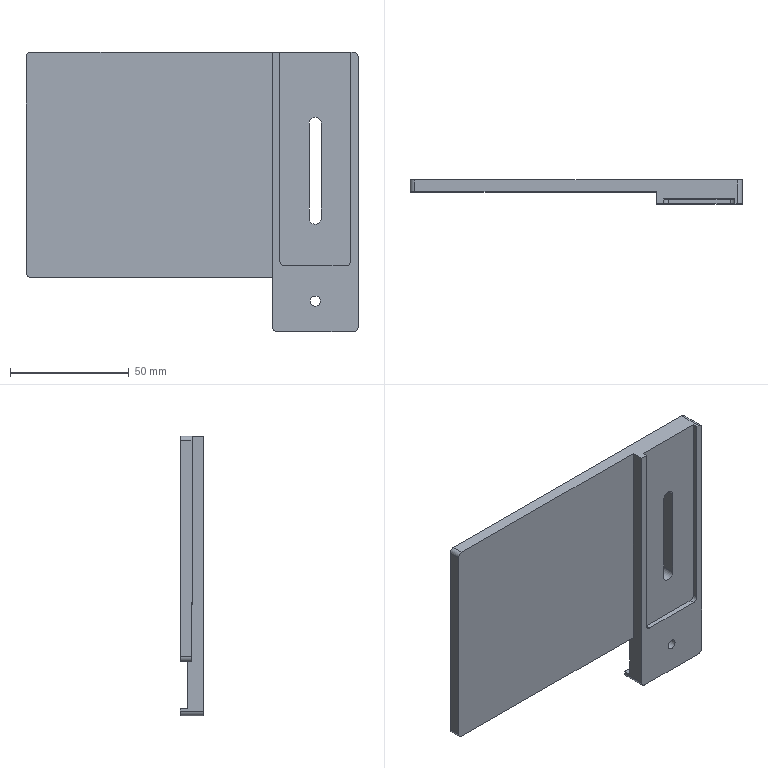Component | SolidWorks | SecondGenerationFour-sidedLabelingTopBatteryPlate-1 | 1 solid | 29 faces | box 140 x 10 x 118 mm | volume 82358 mm3 | plane 18 | cylinder 11 | commonest cylinder face diameters 4 x7 4.2 x2 5.2 x2
build123d program:
from build123d import *

# Parameters (mm, degrees)
SKETCH1_W             = 140
SKETCH1_H             = 95
BOSS_EXTRUDE1_DEPTH   = 10
SKETCH12_W            = 104
SKETCH12_H            = 95
CUT_EXTRUDE2_DEPTH    = 5
CUT_EXTRUDE1_DEPTH    = 86.184
SKETCH13_W            = 36
SKETCH13_H            = 7
BOSS_EXTRUDE3_DEPTH   = 20
M5_TAPPED_HOLE2_D     = 4.2
M5_TAPPED_HOLE2_DEPTH = 20
M5_TAPPED_HOLE2_TIP   = 1.262
SKETCH16_W            = 36
SKETCH16_H            = 10
BOSS_EXTRUDE4_DEPTH   = 3
SKETCH18_W            = 30
SKETCH18_H            = 90
CUT_EXTRUDE4_DEPTH    = 2
FILLET2_R             = 2
FILLET1_R             = 2


with BuildPart() as part:
    # Sketch1 → Boss-Extrude1 (new body)
    with BuildSketch(Plane.XY):
        Rectangle(SKETCH1_W, SKETCH1_H)
    extrude(amount=BOSS_EXTRUDE1_DEPTH)

    # Sketch12 → Cut-Extrude2 (cut)
    with BuildSketch(Plane(origin=(0, 0, 0), x_dir=(-1, 0, 0), z_dir=(0, 0, -1))):
        with Locations((-18, 0)):
            Rectangle(SKETCH12_W, SKETCH12_H)
    extrude(amount=-CUT_EXTRUDE2_DEPTH, mode=Mode.SUBTRACT)

    # Sketch9 → Cut-Extrude1 (cut, through all)
    with BuildSketch(Plane.XY.offset(10)):
        with BuildLine():
            Line((-54.6, -22.5), (-54.6, 17.5))
            ThreePointArc((-54.6, 17.5), (-52, 20.1), (-49.4, 17.5))
            Line((-49.4, 17.5), (-49.4, -22.5))
            ThreePointArc((-49.4, -22.5), (-52, -25.1), (-54.6, -22.5))
        make_face()
    extrude(amount=-CUT_EXTRUDE1_DEPTH, mode=Mode.SUBTRACT)

    # Sketch13 → Boss-Extrude3 (add)
    with BuildSketch(Plane.XZ.offset(47.5)):
        with Locations((-52, 3.5)):
            Rectangle(SKETCH13_W, SKETCH13_H)
    extrude(amount=BOSS_EXTRUDE3_DEPTH)

    # M5 Tapped Hole2
    with Locations(Plane.XY.offset(7)):
        with Locations((-52, -57.5)):
            Hole(M5_TAPPED_HOLE2_D / 2, depth=M5_TAPPED_HOLE2_DEPTH)
            with Locations((0, 0, -(M5_TAPPED_HOLE2_DEPTH + M5_TAPPED_HOLE2_TIP / 2))):  # 118° drill point
                Cone(0, M5_TAPPED_HOLE2_D / 2, M5_TAPPED_HOLE2_TIP, mode=Mode.SUBTRACT)

    # Sketch16 → Boss-Extrude4 (add)
    with BuildSketch(Plane.XZ.offset(67.5)):
        with Locations((-52, 5)):
            Rectangle(SKETCH16_W, SKETCH16_H)
    extrude(amount=BOSS_EXTRUDE4_DEPTH)

    # Sketch18 → Cut-Extrude4 (cut)
    with BuildSketch(Plane(origin=(0, 0, 0), x_dir=(-1, 0, 0), z_dir=(0, 0, -1))):
        with Locations((52, 2.5)):
            Rectangle(SKETCH18_W, SKETCH18_H)
    extrude(amount=-CUT_EXTRUDE4_DEPTH, mode=Mode.SUBTRACT)

    # Fillet2
    fillet2_edges = [part.edges().sort_by_distance(p)[0] for p in [
        (-37, -42.5, 1),
        (-67, -42.5, 1),
    ]]
    fillet(fillet2_edges, radius=FILLET2_R)

    # Fillet1
    fillet1_edges = [part.edges().sort_by_distance(p)[0] for p in [
        (-70, 47.5, 5),
        (70, -47.5, 7.5),
        (70, 47.5, 7.5),
        (-70, -70.5, 5),
        (-34, -70.5, 5),
    ]]
    fillet(fillet1_edges, radius=FILLET1_R)


solid = part.part

# Placed as in the assembly
solid = solid.moved(Location((7.473, 36.863, -79), (-90, 0, 180)))
STEP:
#1=COLOUR_RGB('',0.7922,0.8196,0.9333);
#2=FILL_AREA_STYLE_COLOUR('',#1);
#3=FILL_AREA_STYLE('',(#2));
#4=SURFACE_STYLE_FILL_AREA(#3);
#5=SURFACE_SIDE_STYLE('',(#4));
#6=SURFACE_STYLE_USAGE(.BOTH.,#5);
#7=PRESENTATION_STYLE_ASSIGNMENT((#6));
#8=CARTESIAN_POINT('',(2.259,1.451,-5.374));
#9=VERTEX_POINT('',#8);
#10=CARTESIAN_POINT('',(2.424,1.451,-5.374));
#11=VERTEX_POINT('',#10);
#12=CARTESIAN_POINT('',(2.341,1.451,-5.374));
#13=DIRECTION('',(-0.,-1.,-0.));
#14=DIRECTION('',(1.,0.,0.));
#15=AXIS2_PLACEMENT_3D('',#12,#13,#14);
#16=CIRCLE('',#15,0.08268);
#17=EDGE_CURVE('',#9,#11,#16,.T.);
#18=ORIENTED_EDGE('',*,*,#17,.T.);
#19=CARTESIAN_POINT('',(2.424,1.727,-5.374));
#20=VERTEX_POINT('',#19);
#21=CARTESIAN_POINT('',(2.424,1.727,-5.374));
#22=DIRECTION('',(0.,1.,0.));
#23=VECTOR('',#22,39.37);
#24=LINE('',#21,#23);
#25=EDGE_CURVE('',#11,#20,#24,.T.);
#26=ORIENTED_EDGE('',*,*,#25,.T.);
#27=CARTESIAN_POINT('',(2.259,1.727,-5.374));
#28=VERTEX_POINT('',#27);
#29=CARTESIAN_POINT('',(2.341,1.727,-5.374));
#30=DIRECTION('',(0.,1.,0.));
#31=DIRECTION('',(-1.,0.,0.));
#32=AXIS2_PLACEMENT_3D('',#29,#30,#31);
#33=CIRCLE('',#32,0.08268);
#34=EDGE_CURVE('',#20,#28,#33,.T.);
#35=ORIENTED_EDGE('',*,*,#34,.T.);
#36=CARTESIAN_POINT('',(2.259,1.727,-5.374));
#37=DIRECTION('',(0.,1.,0.));
#38=VECTOR('',#37,39.37);
#39=LINE('',#36,#38);
#40=EDGE_CURVE('',#9,#28,#39,.T.);
#41=ORIENTED_EDGE('',*,*,#40,.F.);
#42=EDGE_LOOP('',(#18,#26,#35,#41));
#43=FACE_OUTER_BOUND('',#42,.T.);
#44=CARTESIAN_POINT('',(2.341,1.727,-5.374));
#45=DIRECTION('',(0.,1.,0.));
#46=DIRECTION('',(-1.,0.,0.));
#47=AXIS2_PLACEMENT_3D('',#44,#45,#46);
#48=CYLINDRICAL_SURFACE('',#47,0.08268);
#49=ADVANCED_FACE('',(#43),#48,.F.);
#50=CARTESIAN_POINT('',(2.444,1.53,-3.996));
#51=VERTEX_POINT('',#50);
#52=CARTESIAN_POINT('',(2.239,1.53,-3.996));
#53=VERTEX_POINT('',#52);
#54=CARTESIAN_POINT('',(2.341,1.53,-3.996));
#55=DIRECTION('',(0.,1.,0.));
#56=DIRECTION('',(1.,0.,0.));
#57=AXIS2_PLACEMENT_3D('',#54,#55,#56);
#58=CIRCLE('',#57,0.1024);
#59=EDGE_CURVE('',#51,#53,#58,.T.);
#60=ORIENTED_EDGE('',*,*,#59,.F.);
#61=CARTESIAN_POINT('',(2.444,1.845,-3.996));
#62=VERTEX_POINT('',#61);
#63=CARTESIAN_POINT('',(2.444,1.451,-3.996));
#64=DIRECTION('',(0.,1.,0.));
#65=VECTOR('',#64,39.37);
#66=LINE('',#63,#65);
#67=EDGE_CURVE('',#51,#62,#66,.T.);
#68=ORIENTED_EDGE('',*,*,#67,.T.);
#69=CARTESIAN_POINT('',(2.239,1.845,-3.996));
#70=VERTEX_POINT('',#69);
#71=CARTESIAN_POINT('',(2.341,1.845,-3.996));
#72=DIRECTION('',(0.,1.,0.));
#73=DIRECTION('',(-1.,0.,0.));
#74=AXIS2_PLACEMENT_3D('',#71,#72,#73);
#75=CIRCLE('',#74,0.1024);
#76=EDGE_CURVE('',#62,#70,#75,.T.);
#77=ORIENTED_EDGE('',*,*,#76,.T.);
#78=CARTESIAN_POINT('',(2.239,1.451,-3.996));
#79=DIRECTION('',(0.,1.,0.));
#80=VECTOR('',#79,39.37);
#81=LINE('',#78,#80);
#82=EDGE_CURVE('',#53,#70,#81,.T.);
#83=ORIENTED_EDGE('',*,*,#82,.F.);
#84=EDGE_LOOP('',(#60,#68,#77,#83));
#85=FACE_OUTER_BOUND('',#84,.T.);
#86=CARTESIAN_POINT('',(2.341,1.451,-3.996));
#87=DIRECTION('',(0.,1.,0.));
#88=DIRECTION('',(-1.,0.,0.));
#89=AXIS2_PLACEMENT_3D('',#86,#87,#88);
#90=CYLINDRICAL_SURFACE('',#89,0.1024);
#91=ADVANCED_FACE('',(#85),#90,.F.);
#92=CARTESIAN_POINT('',(2.444,1.53,-2.421));
#93=VERTEX_POINT('',#92);
#94=CARTESIAN_POINT('',(2.444,1.53,-3.996));
#95=DIRECTION('',(-0.,0.,-1.));
#96=VECTOR('',#95,39.37);
#97=LINE('',#94,#96);
#98=EDGE_CURVE('',#93,#51,#97,.T.);
#99=ORIENTED_EDGE('',*,*,#98,.F.);
#100=CARTESIAN_POINT('',(2.444,1.845,-2.421));
#101=VERTEX_POINT('',#100);
#102=CARTESIAN_POINT('',(2.444,1.451,-2.421));
#103=DIRECTION('',(0.,1.,0.));
#104=VECTOR('',#103,39.37);
#105=LINE('',#102,#104);
#106=EDGE_CURVE('',#93,#101,#105,.T.);
#107=ORIENTED_EDGE('',*,*,#106,.T.);
#108=CARTESIAN_POINT('',(2.444,1.845,-3.996));
#109=DIRECTION('',(-0.,0.,-1.));
#110=VECTOR('',#109,39.37);
#111=LINE('',#108,#110);
#112=EDGE_CURVE('',#101,#62,#111,.T.);
#113=ORIENTED_EDGE('',*,*,#112,.T.);
#114=ORIENTED_EDGE('',*,*,#67,.F.);
#115=EDGE_LOOP('',(#99,#107,#113,#114));
#116=FACE_OUTER_BOUND('',#115,.T.);
#117=CARTESIAN_POINT('',(2.444,1.451,-3.996));
#118=DIRECTION('',(1.,-0.,-0.));
#119=DIRECTION('',(-0.,0.,-1.));
#120=AXIS2_PLACEMENT_3D('',#117,#118,#119);
#121=PLANE('',#120);
#122=ADVANCED_FACE('',(#116),#121,.F.);
#123=CARTESIAN_POINT('',(2.239,1.53,-2.421));
#124=VERTEX_POINT('',#123);
#125=CARTESIAN_POINT('',(2.341,1.53,-2.421));
#126=DIRECTION('',(0.,1.,0.));
#127=DIRECTION('',(1.,0.,0.));
#128=AXIS2_PLACEMENT_3D('',#125,#126,#127);
#129=CIRCLE('',#128,0.1024);
#130=EDGE_CURVE('',#124,#93,#129,.T.);
#131=ORIENTED_EDGE('',*,*,#130,.F.);
#132=CARTESIAN_POINT('',(2.239,1.845,-2.421));
#133=VERTEX_POINT('',#132);
#134=CARTESIAN_POINT('',(2.239,1.451,-2.421));
#135=DIRECTION('',(0.,1.,0.));
#136=VECTOR('',#135,39.37);
#137=LINE('',#134,#136);
#138=EDGE_CURVE('',#124,#133,#137,.T.);
#139=ORIENTED_EDGE('',*,*,#138,.T.);
#140=CARTESIAN_POINT('',(2.341,1.845,-2.421));
#141=DIRECTION('',(0.,1.,0.));
#142=DIRECTION('',(-1.,0.,0.));
#143=AXIS2_PLACEMENT_3D('',#140,#141,#142);
#144=CIRCLE('',#143,0.1024);
#145=EDGE_CURVE('',#133,#101,#144,.T.);
#146=ORIENTED_EDGE('',*,*,#145,.T.);
#147=ORIENTED_EDGE('',*,*,#106,.F.);
#148=EDGE_LOOP('',(#131,#139,#146,#147));
#149=FACE_OUTER_BOUND('',#148,.T.);
#150=CARTESIAN_POINT('',(2.341,1.451,-2.421));
#151=DIRECTION('',(0.,1.,0.));
#152=DIRECTION('',(-1.,0.,0.));
#153=AXIS2_PLACEMENT_3D('',#150,#151,#152);
#154=CYLINDRICAL_SURFACE('',#153,0.1024);
#155=ADVANCED_FACE('',(#149),#154,.F.);
#156=CARTESIAN_POINT('',(2.239,1.53,-3.996));
#157=DIRECTION('',(0.,-0.,1.));
#158=VECTOR('',#157,39.37);
#159=LINE('',#156,#158);
#160=EDGE_CURVE('',#53,#124,#159,.T.);
#161=ORIENTED_EDGE('',*,*,#160,.F.);
#162=ORIENTED_EDGE('',*,*,#82,.T.);
#163=CARTESIAN_POINT('',(2.239,1.845,-3.996));
#164=DIRECTION('',(0.,-0.,1.));
#165=VECTOR('',#164,39.37);
#166=LINE('',#163,#165);
#167=EDGE_CURVE('',#70,#133,#166,.T.);
#168=ORIENTED_EDGE('',*,*,#167,.T.);
#169=ORIENTED_EDGE('',*,*,#138,.F.);
#170=EDGE_LOOP('',(#161,#162,#168,#169));
#171=FACE_OUTER_BOUND('',#170,.T.);
#172=CARTESIAN_POINT('',(2.239,1.451,-3.996));
#173=DIRECTION('',(-1.,0.,0.));
#174=DIRECTION('',(0.,-0.,1.));
#175=AXIS2_PLACEMENT_3D('',#172,#173,#174);
#176=PLANE('',#175);
#177=ADVANCED_FACE('',(#171),#176,.F.);
#178=CARTESIAN_POINT('',(-2.383,1.648,-4.98));
#179=VERTEX_POINT('',#178);
#180=CARTESIAN_POINT('',(1.633,1.648,-4.98));
#181=VERTEX_POINT('',#180);
#182=CARTESIAN_POINT('',(-2.462,1.648,-4.98));
#183=DIRECTION('',(1.,-0.,-0.));
#184=VECTOR('',#183,39.37);
#185=LINE('',#182,#184);
#186=EDGE_CURVE('',#179,#181,#185,.T.);
#187=ORIENTED_EDGE('',*,*,#186,.F.);
#188=CARTESIAN_POINT('',(-2.383,1.845,-4.98));
#189=VERTEX_POINT('',#188);
#190=CARTESIAN_POINT('',(-2.383,1.845,-4.98));
#191=DIRECTION('',(0.,1.,0.));
#192=VECTOR('',#191,39.37);
#193=LINE('',#190,#192);
#194=EDGE_CURVE('',#179,#189,#193,.T.);
#195=ORIENTED_EDGE('',*,*,#194,.T.);
#196=CARTESIAN_POINT('',(3.05,1.845,-4.98));
#197=VERTEX_POINT('',#196);
#198=CARTESIAN_POINT('',(3.05,1.845,-4.98));
#199=DIRECTION('',(-1.,0.,0.));
#200=VECTOR('',#199,39.37);
#201=LINE('',#198,#200);
#202=EDGE_CURVE('',#197,#189,#201,.T.);
#203=ORIENTED_EDGE('',*,*,#202,.F.);
#204=CARTESIAN_POINT('',(3.05,1.727,-4.98));
#205=VERTEX_POINT('',#204);
#206=CARTESIAN_POINT('',(3.05,1.845,-4.98));
#207=DIRECTION('',(-0.,-1.,-0.));
#208=VECTOR('',#207,39.37);
#209=LINE('',#206,#208);
#210=EDGE_CURVE('',#197,#205,#209,.T.);
#211=ORIENTED_EDGE('',*,*,#210,.T.);
#212=CARTESIAN_POINT('',(1.633,1.727,-4.98));
#213=VERTEX_POINT('',#212);
#214=CARTESIAN_POINT('',(1.633,1.727,-4.98));
#215=DIRECTION('',(1.,-0.,-0.));
#216=VECTOR('',#215,39.37);
#217=LINE('',#214,#216);
#218=EDGE_CURVE('',#213,#205,#217,.T.);
#219=ORIENTED_EDGE('',*,*,#218,.F.);
#220=CARTESIAN_POINT('',(1.633,1.451,-4.98));
#221=DIRECTION('',(0.,1.,0.));
#222=VECTOR('',#221,39.37);
#223=LINE('',#220,#222);
#224=EDGE_CURVE('',#181,#213,#223,.T.);
#225=ORIENTED_EDGE('',*,*,#224,.F.);
#226=EDGE_LOOP('',(#187,#195,#203,#211,#219,#225));
#227=FACE_OUTER_BOUND('',#226,.T.);
#228=CARTESIAN_POINT('',(3.05,1.845,-4.98));
#229=DIRECTION('',(0.,-0.,1.));
#230=DIRECTION('',(0.,1.,0.));
#231=AXIS2_PLACEMENT_3D('',#228,#229,#230);
#232=PLANE('',#231);
#233=ADVANCED_FACE('',(#227),#232,.F.);
#234=CARTESIAN_POINT('',(-2.462,1.845,-4.902));
#235=VERTEX_POINT('',#234);
#236=CARTESIAN_POINT('',(-2.462,1.845,-1.319));
#237=VERTEX_POINT('',#236);
#238=CARTESIAN_POINT('',(-2.462,1.845,-4.98));
#239=DIRECTION('',(0.,-0.,1.));
#240=VECTOR('',#239,39.37);
#241=LINE('',#238,#240);
#242=EDGE_CURVE('',#235,#237,#241,.T.);
#243=ORIENTED_EDGE('',*,*,#242,.F.);
#244=CARTESIAN_POINT('',(-2.462,1.648,-4.902));
#245=VERTEX_POINT('',#244);
#246=CARTESIAN_POINT('',(-2.462,1.845,-4.902));
#247=DIRECTION('',(-0.,-1.,-0.));
#248=VECTOR('',#247,39.37);
#249=LINE('',#246,#248);
#250=EDGE_CURVE('',#235,#245,#249,.T.);
#251=ORIENTED_EDGE('',*,*,#250,.T.);
#252=CARTESIAN_POINT('',(-2.462,1.648,-1.319));
#253=VERTEX_POINT('',#252);
#254=CARTESIAN_POINT('',(-2.462,1.648,-1.24));
#255=DIRECTION('',(-0.,0.,-1.));
#256=VECTOR('',#255,39.37);
#257=LINE('',#254,#256);
#258=EDGE_CURVE('',#253,#245,#257,.T.);
#259=ORIENTED_EDGE('',*,*,#258,.F.);
#260=CARTESIAN_POINT('',(-2.462,1.845,-1.319));
#261=DIRECTION('',(0.,1.,0.));
#262=VECTOR('',#261,39.37);
#263=LINE('',#260,#262);
#264=EDGE_CURVE('',#253,#237,#263,.T.);
#265=ORIENTED_EDGE('',*,*,#264,.T.);
#266=EDGE_LOOP('',(#243,#251,#259,#265));
#267=FACE_OUTER_BOUND('',#266,.T.);
#268=CARTESIAN_POINT('',(-2.462,1.845,-4.98));
#269=DIRECTION('',(1.,-0.,-0.));
#270=DIRECTION('',(0.,1.,0.));
#271=AXIS2_PLACEMENT_3D('',#268,#269,#270);
#272=PLANE('',#271);
#273=ADVANCED_FACE('',(#267),#272,.F.);
#274=CARTESIAN_POINT('',(2.932,1.451,-1.24));
#275=VERTEX_POINT('',#274);
#276=CARTESIAN_POINT('',(2.971,1.451,-1.24));
#277=VERTEX_POINT('',#276);
#278=CARTESIAN_POINT('',(3.05,1.451,-1.24));
#279=DIRECTION('',(1.,-0.,-0.));
#280=VECTOR('',#279,39.37);
#281=LINE('',#278,#280);
#282=EDGE_CURVE('',#275,#277,#281,.T.);
#283=ORIENTED_EDGE('',*,*,#282,.T.);
#284=CARTESIAN_POINT('',(2.971,1.845,-1.24));
#285=VERTEX_POINT('',#284);
#286=CARTESIAN_POINT('',(2.971,1.845,-1.24));
#287=DIRECTION('',(0.,1.,0.));
#288=VECTOR('',#287,39.37);
#289=LINE('',#286,#288);
#290=EDGE_CURVE('',#277,#285,#289,.T.);
#291=ORIENTED_EDGE('',*,*,#290,.T.);
#292=CARTESIAN_POINT('',(-2.383,1.845,-1.24));
#293=VERTEX_POINT('',#292);
#294=CARTESIAN_POINT('',(3.05,1.845,-1.24));
#295=DIRECTION('',(1.,-0.,-0.));
#296=VECTOR('',#295,39.37);
#297=LINE('',#294,#296);
#298=EDGE_CURVE('',#293,#285,#297,.T.);
#299=ORIENTED_EDGE('',*,*,#298,.F.);
#300=CARTESIAN_POINT('',(-2.383,1.648,-1.24));
#301=VERTEX_POINT('',#300);
#302=CARTESIAN_POINT('',(-2.383,1.845,-1.24));
#303=DIRECTION('',(-0.,-1.,-0.));
#304=VECTOR('',#303,39.37);
#305=LINE('',#302,#304);
#306=EDGE_CURVE('',#293,#301,#305,.T.);
#307=ORIENTED_EDGE('',*,*,#306,.T.);
#308=CARTESIAN_POINT('',(1.633,1.648,-1.24));
#309=VERTEX_POINT('',#308);
#310=CARTESIAN_POINT('',(-2.462,1.648,-1.24));
#311=DIRECTION('',(-1.,0.,0.));
#312=VECTOR('',#311,39.37);
#313=LINE('',#310,#312);
#314=EDGE_CURVE('',#309,#301,#313,.T.);
#315=ORIENTED_EDGE('',*,*,#314,.F.);
#316=CARTESIAN_POINT('',(1.633,1.451,-1.24));
#317=VERTEX_POINT('',#316);
#318=CARTESIAN_POINT('',(1.633,1.648,-1.24));
#319=DIRECTION('',(-0.,-1.,-0.));
#320=VECTOR('',#319,39.37);
#321=LINE('',#318,#320);
#322=EDGE_CURVE('',#309,#317,#321,.T.);
#323=ORIENTED_EDGE('',*,*,#322,.T.);
#324=CARTESIAN_POINT('',(1.751,1.451,-1.24));
#325=VERTEX_POINT('',#324);
#326=CARTESIAN_POINT('',(3.05,1.451,-1.24));
#327=DIRECTION('',(1.,-0.,-0.));
#328=VECTOR('',#327,39.37);
#329=LINE('',#326,#328);
#330=EDGE_CURVE('',#317,#325,#329,.T.);
#331=ORIENTED_EDGE('',*,*,#330,.T.);
#332=CARTESIAN_POINT('',(1.751,1.53,-1.24));
#333=VERTEX_POINT('',#332);
#334=CARTESIAN_POINT('',(1.751,1.53,-1.24));
#335=DIRECTION('',(-0.,-1.,-0.));
#336=VECTOR('',#335,39.37);
#337=LINE('',#334,#336);
#338=EDGE_CURVE('',#333,#325,#337,.T.);
#339=ORIENTED_EDGE('',*,*,#338,.F.);
#340=CARTESIAN_POINT('',(2.932,1.53,-1.24));
#341=VERTEX_POINT('',#340);
#342=CARTESIAN_POINT('',(1.751,1.53,-1.24));
#343=DIRECTION('',(-1.,0.,0.));
#344=VECTOR('',#343,39.37);
#345=LINE('',#342,#344);
#346=EDGE_CURVE('',#341,#333,#345,.T.);
#347=ORIENTED_EDGE('',*,*,#346,.F.);
#348=CARTESIAN_POINT('',(2.932,1.53,-1.24));
#349=DIRECTION('',(-0.,-1.,-0.));
#350=VECTOR('',#349,39.37);
#351=LINE('',#348,#350);
#352=EDGE_CURVE('',#341,#275,#351,.T.);
#353=ORIENTED_EDGE('',*,*,#352,.T.);
#354=EDGE_LOOP('',(#283,#291,#299,#307,#315,#323,#331,#339,#347,#353));
#355=FACE_OUTER_BOUND('',#354,.T.);
#356=CARTESIAN_POINT('',(3.05,1.845,-1.24));
#357=DIRECTION('',(-0.,0.,-1.));
#358=DIRECTION('',(-0.,-1.,-0.));
#359=AXIS2_PLACEMENT_3D('',#356,#357,#358);
#360=PLANE('',#359);
#361=ADVANCED_FACE('',(#355),#360,.F.);
#362=CARTESIAN_POINT('',(3.05,1.451,-1.319));
#363=VERTEX_POINT('',#362);
#364=CARTESIAN_POINT('',(3.05,1.451,-5.807));
#365=VERTEX_POINT('',#364);
#366=CARTESIAN_POINT('',(3.05,1.451,-4.98));
#367=DIRECTION('',(-0.,0.,-1.));
#368=VECTOR('',#367,39.37);
#369=LINE('',#366,#368);
#370=EDGE_CURVE('',#363,#365,#369,.T.);
#371=ORIENTED_EDGE('',*,*,#370,.T.);
#372=CARTESIAN_POINT('',(3.05,1.845,-5.807));
#373=VERTEX_POINT('',#372);
#374=CARTESIAN_POINT('',(3.05,1.845,-5.807));
#375=DIRECTION('',(0.,1.,0.));
#376=VECTOR('',#375,39.37);
#377=LINE('',#374,#376);
#378=EDGE_CURVE('',#365,#373,#377,.T.);
#379=ORIENTED_EDGE('',*,*,#378,.T.);
#380=CARTESIAN_POINT('',(3.05,1.845,-5.768));
#381=VERTEX_POINT('',#380);
#382=CARTESIAN_POINT('',(3.05,1.845,-5.886));
#383=DIRECTION('',(0.,-0.,1.));
#384=VECTOR('',#383,39.37);
#385=LINE('',#382,#384);
#386=EDGE_CURVE('',#373,#381,#385,.T.);
#387=ORIENTED_EDGE('',*,*,#386,.T.);
#388=CARTESIAN_POINT('',(3.05,1.727,-5.768));
#389=VERTEX_POINT('',#388);
#390=CARTESIAN_POINT('',(3.05,1.451,-5.768));
#391=DIRECTION('',(-0.,-1.,-0.));
#392=VECTOR('',#391,39.37);
#393=LINE('',#390,#392);
#394=EDGE_CURVE('',#381,#389,#393,.T.);
#395=ORIENTED_EDGE('',*,*,#394,.T.);
#396=CARTESIAN_POINT('',(3.05,1.727,-5.768));
#397=DIRECTION('',(0.,-0.,1.));
#398=VECTOR('',#397,39.37);
#399=LINE('',#396,#398);
#400=EDGE_CURVE('',#389,#205,#399,.T.);
#401=ORIENTED_EDGE('',*,*,#400,.T.);
#402=ORIENTED_EDGE('',*,*,#210,.F.);
#403=CARTESIAN_POINT('',(3.05,1.845,-1.319));
#404=VERTEX_POINT('',#403);
#405=CARTESIAN_POINT('',(3.05,1.845,-4.98));
#406=DIRECTION('',(-0.,0.,-1.));
#407=VECTOR('',#406,39.37);
#408=LINE('',#405,#407);
#409=EDGE_CURVE('',#404,#197,#408,.T.);
#410=ORIENTED_EDGE('',*,*,#409,.F.);
#411=CARTESIAN_POINT('',(3.05,1.845,-1.319));
#412=DIRECTION('',(-0.,-1.,-0.));
#413=VECTOR('',#412,39.37);
#414=LINE('',#411,#413);
#415=EDGE_CURVE('',#404,#363,#414,.T.);
#416=ORIENTED_EDGE('',*,*,#415,.T.);
#417=EDGE_LOOP('',(#371,#379,#387,#395,#401,#402,#410,#416));
#418=FACE_OUTER_BOUND('',#417,.T.);
#419=CARTESIAN_POINT('',(3.05,1.845,-4.98));
#420=DIRECTION('',(-1.,0.,0.));
#421=DIRECTION('',(-0.,-1.,-0.));
#422=AXIS2_PLACEMENT_3D('',#419,#420,#421);
#423=PLANE('',#422);
#424=ADVANCED_FACE('',(#418),#423,.F.);
#425=ORIENTED_EDGE('',*,*,#167,.F.);
#426=ORIENTED_EDGE('',*,*,#76,.F.);
#427=ORIENTED_EDGE('',*,*,#112,.F.);
#428=ORIENTED_EDGE('',*,*,#145,.F.);
#429=EDGE_LOOP('',(#425,#426,#427,#428));
#430=FACE_BOUND('',#429,.T.);
#431=ORIENTED_EDGE('',*,*,#298,.T.);
#432=CARTESIAN_POINT('',(2.971,1.845,-1.319));
#433=DIRECTION('',(0.,1.,0.));
#434=DIRECTION('',(1.,0.,0.));
#435=AXIS2_PLACEMENT_3D('',#432,#433,#434);
#436=CIRCLE('',#435,0.07874);
#437=EDGE_CURVE('',#285,#404,#436,.T.);
#438=ORIENTED_EDGE('',*,*,#437,.T.);
#439=ORIENTED_EDGE('',*,*,#409,.T.);
#440=ORIENTED_EDGE('',*,*,#202,.T.);
#441=CARTESIAN_POINT('',(-2.383,1.845,-4.902));
#442=DIRECTION('',(0.,1.,0.));
#443=DIRECTION('',(1.,0.,0.));
#444=AXIS2_PLACEMENT_3D('',#441,#442,#443);
#445=CIRCLE('',#444,0.07874);
#446=EDGE_CURVE('',#189,#235,#445,.T.);
#447=ORIENTED_EDGE('',*,*,#446,.T.);
#448=ORIENTED_EDGE('',*,*,#242,.T.);
#449=CARTESIAN_POINT('',(-2.383,1.845,-1.319));
#450=DIRECTION('',(0.,1.,0.));
#451=DIRECTION('',(1.,0.,0.));
#452=AXIS2_PLACEMENT_3D('',#449,#450,#451);
#453=CIRCLE('',#452,0.07874);
#454=EDGE_CURVE('',#237,#293,#453,.T.);
#455=ORIENTED_EDGE('',*,*,#454,.T.);
#456=EDGE_LOOP('',(#431,#438,#439,#440,#447,#448,#455));
#457=FACE_OUTER_BOUND('',#456,.T.);
#458=CARTESIAN_POINT('',(-2.462,1.845,-1.24));
#459=DIRECTION('',(-0.,-1.,-0.));
#460=DIRECTION('',(1.,-0.,-0.));
#461=AXIS2_PLACEMENT_3D('',#458,#459,#460);
#462=PLANE('',#461);
#463=ADVANCED_FACE('',(#430,#457),#462,.F.);
#464=CARTESIAN_POINT('',(2.971,1.451,-5.886));
#465=VERTEX_POINT('',#464);
#466=CARTESIAN_POINT('',(1.712,1.451,-5.886));
#467=VERTEX_POINT('',#466);
#468=CARTESIAN_POINT('',(3.05,1.451,-5.886));
#469=DIRECTION('',(-1.,0.,0.));
#470=VECTOR('',#469,39.37);
#471=LINE('',#468,#470);
#472=EDGE_CURVE('',#465,#467,#471,.T.);
#473=ORIENTED_EDGE('',*,*,#472,.F.);
#474=CARTESIAN_POINT('',(2.971,1.451,-5.807));
#475=DIRECTION('',(-0.,-1.,-0.));
#476=DIRECTION('',(1.,0.,0.));
#477=AXIS2_PLACEMENT_3D('',#474,#475,#476);
#478=CIRCLE('',#477,0.07874);
#479=EDGE_CURVE('',#465,#365,#478,.T.);
#480=ORIENTED_EDGE('',*,*,#479,.T.);
#481=ORIENTED_EDGE('',*,*,#370,.F.);
#482=CARTESIAN_POINT('',(2.971,1.451,-1.319));
#483=DIRECTION('',(-0.,-1.,-0.));
#484=DIRECTION('',(1.,0.,0.));
#485=AXIS2_PLACEMENT_3D('',#482,#483,#484);
#486=CIRCLE('',#485,0.07874);
#487=EDGE_CURVE('',#363,#277,#486,.T.);
#488=ORIENTED_EDGE('',*,*,#487,.T.);
#489=ORIENTED_EDGE('',*,*,#282,.F.);
#490=CARTESIAN_POINT('',(2.932,1.451,-4.705));
#491=VERTEX_POINT('',#490);
#492=CARTESIAN_POINT('',(2.932,1.451,-1.24));
#493=DIRECTION('',(0.,-0.,1.));
#494=VECTOR('',#493,39.37);
#495=LINE('',#492,#494);
#496=EDGE_CURVE('',#491,#275,#495,.T.);
#497=ORIENTED_EDGE('',*,*,#496,.F.);
#498=CARTESIAN_POINT('',(2.853,1.451,-4.783));
#499=VERTEX_POINT('',#498);
#500=CARTESIAN_POINT('',(2.853,1.451,-4.705));
#501=DIRECTION('',(0.,1.,0.));
#502=DIRECTION('',(1.,0.,0.));
#503=AXIS2_PLACEMENT_3D('',#500,#501,#502);
#504=CIRCLE('',#503,0.07874);
#505=EDGE_CURVE('',#491,#499,#504,.T.);
#506=ORIENTED_EDGE('',*,*,#505,.T.);
#507=CARTESIAN_POINT('',(1.83,1.451,-4.783));
#508=VERTEX_POINT('',#507);
#509=CARTESIAN_POINT('',(1.751,1.451,-4.783));
#510=DIRECTION('',(1.,-0.,-0.));
#511=VECTOR('',#510,39.37);
#512=LINE('',#509,#511);
#513=EDGE_CURVE('',#508,#499,#512,.T.);
#514=ORIENTED_EDGE('',*,*,#513,.F.);
#515=CARTESIAN_POINT('',(1.751,1.451,-4.705));
#516=VERTEX_POINT('',#515);
#517=CARTESIAN_POINT('',(1.83,1.451,-4.705));
#518=DIRECTION('',(0.,1.,0.));
#519=DIRECTION('',(1.,0.,0.));
#520=AXIS2_PLACEMENT_3D('',#517,#518,#519);
#521=CIRCLE('',#520,0.07874);
#522=EDGE_CURVE('',#508,#516,#521,.T.);
#523=ORIENTED_EDGE('',*,*,#522,.T.);
#524=CARTESIAN_POINT('',(1.751,1.451,-1.24));
#525=DIRECTION('',(0.,0.,-1.));
#526=VECTOR('',#525,39.37);
#527=LINE('',#524,#526);
#528=EDGE_CURVE('',#325,#516,#527,.T.);
#529=ORIENTED_EDGE('',*,*,#528,.F.);
#530=ORIENTED_EDGE('',*,*,#330,.F.);
#531=CARTESIAN_POINT('',(1.633,1.451,-5.807));
#532=VERTEX_POINT('',#531);
#533=CARTESIAN_POINT('',(1.633,1.451,-1.24));
#534=DIRECTION('',(0.,-0.,1.));
#535=VECTOR('',#534,39.37);
#536=LINE('',#533,#535);
#537=EDGE_CURVE('',#532,#317,#536,.T.);
#538=ORIENTED_EDGE('',*,*,#537,.F.);
#539=CARTESIAN_POINT('',(1.712,1.451,-5.807));
#540=DIRECTION('',(-0.,-1.,-0.));
#541=DIRECTION('',(1.,0.,0.));
#542=AXIS2_PLACEMENT_3D('',#539,#540,#541);
#543=CIRCLE('',#542,0.07874);
#544=EDGE_CURVE('',#532,#467,#543,.T.);
#545=ORIENTED_EDGE('',*,*,#544,.T.);
#546=EDGE_LOOP('',(#473,#480,#481,#488,#489,#497,#506,#514,#523,#529,#530,#538,#545));
#547=FACE_OUTER_BOUND('',#546,.T.);
#548=ORIENTED_EDGE('',*,*,#17,.F.);
#549=CARTESIAN_POINT('',(2.341,1.451,-5.374));
#550=DIRECTION('',(-0.,-1.,-0.));
#551=DIRECTION('',(1.,0.,0.));
#552=AXIS2_PLACEMENT_3D('',#549,#550,#551);
#553=CIRCLE('',#552,0.08268);
#554=EDGE_CURVE('',#11,#9,#553,.T.);
#555=ORIENTED_EDGE('',*,*,#554,.F.);
#556=EDGE_LOOP('',(#548,#555));
#557=FACE_BOUND('',#556,.T.);
#558=CARTESIAN_POINT('',(-2.462,1.451,-1.24));
#559=DIRECTION('',(-0.,-1.,-0.));
#560=DIRECTION('',(1.,-0.,-0.));
#561=AXIS2_PLACEMENT_3D('',#558,#559,#560);
#562=PLANE('',#561);
#563=ADVANCED_FACE('',(#547,#557),#562,.T.);
#564=CARTESIAN_POINT('',(1.633,1.845,-5.807));
#565=VERTEX_POINT('',#564);
#566=CARTESIAN_POINT('',(1.633,1.845,-5.768));
#567=VERTEX_POINT('',#566);
#568=CARTESIAN_POINT('',(1.633,1.845,-5.886));
#569=DIRECTION('',(0.,-0.,1.));
#570=VECTOR('',#569,39.37);
#571=LINE('',#568,#570);
#572=EDGE_CURVE('',#565,#567,#571,.T.);
#573=ORIENTED_EDGE('',*,*,#572,.F.);
#574=CARTESIAN_POINT('',(1.633,1.648,-5.807));
#575=DIRECTION('',(-0.,-1.,-0.));
#576=VECTOR('',#575,39.37);
#577=LINE('',#574,#576);
#578=EDGE_CURVE('',#565,#532,#577,.T.);
#579=ORIENTED_EDGE('',*,*,#578,.T.);
#580=ORIENTED_EDGE('',*,*,#537,.T.);
#581=ORIENTED_EDGE('',*,*,#322,.F.);
#582=CARTESIAN_POINT('',(1.633,1.648,-1.24));
#583=DIRECTION('',(0.,-0.,1.));
#584=VECTOR('',#583,39.37);
#585=LINE('',#582,#584);
#586=EDGE_CURVE('',#181,#309,#585,.T.);
#587=ORIENTED_EDGE('',*,*,#586,.F.);
#588=ORIENTED_EDGE('',*,*,#224,.T.);
#589=CARTESIAN_POINT('',(1.633,1.727,-5.768));
#590=VERTEX_POINT('',#589);
#591=CARTESIAN_POINT('',(1.633,1.727,-5.768));
#592=DIRECTION('',(0.,-0.,1.));
#593=VECTOR('',#592,39.37);
#594=LINE('',#591,#593);
#595=EDGE_CURVE('',#590,#213,#594,.T.);
#596=ORIENTED_EDGE('',*,*,#595,.F.);
#597=CARTESIAN_POINT('',(1.633,1.451,-5.768));
#598=DIRECTION('',(0.,1.,0.));
#599=VECTOR('',#598,39.37);
#600=LINE('',#597,#599);
#601=EDGE_CURVE('',#590,#567,#600,.T.);
#602=ORIENTED_EDGE('',*,*,#601,.T.);
#603=EDGE_LOOP('',(#573,#579,#580,#581,#587,#588,#596,#602));
#604=FACE_OUTER_BOUND('',#603,.T.);
#605=CARTESIAN_POINT('',(1.633,1.648,-1.24));
#606=DIRECTION('',(1.,-0.,-0.));
#607=DIRECTION('',(0.,1.,0.));
#608=AXIS2_PLACEMENT_3D('',#605,#606,#607);
#609=PLANE('',#608);
#610=ADVANCED_FACE('',(#604),#609,.F.);
#611=ORIENTED_EDGE('',*,*,#258,.T.);
#612=CARTESIAN_POINT('',(-2.383,1.648,-4.902));
#613=DIRECTION('',(-0.,-1.,-0.));
#614=DIRECTION('',(1.,0.,0.));
#615=AXIS2_PLACEMENT_3D('',#612,#613,#614);
#616=CIRCLE('',#615,0.07874);
#617=EDGE_CURVE('',#245,#179,#616,.T.);
#618=ORIENTED_EDGE('',*,*,#617,.T.);
#619=ORIENTED_EDGE('',*,*,#186,.T.);
#620=ORIENTED_EDGE('',*,*,#586,.T.);
#621=ORIENTED_EDGE('',*,*,#314,.T.);
#622=CARTESIAN_POINT('',(-2.383,1.648,-1.319));
#623=DIRECTION('',(-0.,-1.,-0.));
#624=DIRECTION('',(1.,0.,0.));
#625=AXIS2_PLACEMENT_3D('',#622,#623,#624);
#626=CIRCLE('',#625,0.07874);
#627=EDGE_CURVE('',#301,#253,#626,.T.);
#628=ORIENTED_EDGE('',*,*,#627,.T.);
#629=EDGE_LOOP('',(#611,#618,#619,#620,#621,#628));
#630=FACE_OUTER_BOUND('',#629,.T.);
#631=CARTESIAN_POINT('',(-2.462,1.648,-4.98));
#632=DIRECTION('',(-0.,-1.,-0.));
#633=DIRECTION('',(1.,-0.,-0.));
#634=AXIS2_PLACEMENT_3D('',#631,#632,#633);
#635=PLANE('',#634);
#636=ADVANCED_FACE('',(#630),#635,.T.);
#637=CARTESIAN_POINT('',(2.341,1.727,-5.374));
#638=DIRECTION('',(0.,1.,0.));
#639=DIRECTION('',(-1.,0.,0.));
#640=AXIS2_PLACEMENT_3D('',#637,#638,#639);
#641=CIRCLE('',#640,0.08268);
#642=EDGE_CURVE('',#28,#20,#641,.T.);
#643=ORIENTED_EDGE('',*,*,#642,.F.);
#644=ORIENTED_EDGE('',*,*,#34,.F.);
#645=EDGE_LOOP('',(#643,#644));
#646=FACE_BOUND('',#645,.T.);
#647=ORIENTED_EDGE('',*,*,#218,.T.);
#648=ORIENTED_EDGE('',*,*,#400,.F.);
#649=CARTESIAN_POINT('',(1.633,1.727,-5.768));
#650=DIRECTION('',(1.,-0.,-0.));
#651=VECTOR('',#650,39.37);
#652=LINE('',#649,#651);
#653=EDGE_CURVE('',#590,#389,#652,.T.);
#654=ORIENTED_EDGE('',*,*,#653,.F.);
#655=ORIENTED_EDGE('',*,*,#595,.T.);
#656=EDGE_LOOP('',(#647,#648,#654,#655));
#657=FACE_OUTER_BOUND('',#656,.T.);
#658=CARTESIAN_POINT('',(1.633,1.727,-5.768));
#659=DIRECTION('',(-0.,-1.,-0.));
#660=DIRECTION('',(1.,-0.,-0.));
#661=AXIS2_PLACEMENT_3D('',#658,#659,#660);
#662=PLANE('',#661);
#663=ADVANCED_FACE('',(#646,#657),#662,.F.);
#664=ORIENTED_EDGE('',*,*,#25,.F.);
#665=ORIENTED_EDGE('',*,*,#554,.T.);
#666=ORIENTED_EDGE('',*,*,#40,.T.);
#667=ORIENTED_EDGE('',*,*,#642,.T.);
#668=EDGE_LOOP('',(#664,#665,#666,#667));
#669=FACE_OUTER_BOUND('',#668,.T.);
#670=CARTESIAN_POINT('',(2.341,1.727,-5.374));
#671=DIRECTION('',(0.,1.,0.));
#672=DIRECTION('',(-1.,0.,0.));
#673=AXIS2_PLACEMENT_3D('',#670,#671,#672);
#674=CYLINDRICAL_SURFACE('',#673,0.08268);
#675=ADVANCED_FACE('',(#669),#674,.F.);
#676=ORIENTED_EDGE('',*,*,#386,.F.);
#677=CARTESIAN_POINT('',(2.971,1.845,-5.886));
#678=VERTEX_POINT('',#677);
#679=CARTESIAN_POINT('',(2.971,1.845,-5.807));
#680=DIRECTION('',(0.,1.,0.));
#681=DIRECTION('',(1.,0.,0.));
#682=AXIS2_PLACEMENT_3D('',#679,#680,#681);
#683=CIRCLE('',#682,0.07874);
#684=EDGE_CURVE('',#373,#678,#683,.T.);
#685=ORIENTED_EDGE('',*,*,#684,.T.);
#686=CARTESIAN_POINT('',(1.712,1.845,-5.886));
#687=VERTEX_POINT('',#686);
#688=CARTESIAN_POINT('',(3.05,1.845,-5.886));
#689=DIRECTION('',(1.,-0.,-0.));
#690=VECTOR('',#689,39.37);
#691=LINE('',#688,#690);
#692=EDGE_CURVE('',#687,#678,#691,.T.);
#693=ORIENTED_EDGE('',*,*,#692,.F.);
#694=CARTESIAN_POINT('',(1.712,1.845,-5.807));
#695=DIRECTION('',(0.,1.,0.));
#696=DIRECTION('',(1.,0.,0.));
#697=AXIS2_PLACEMENT_3D('',#694,#695,#696);
#698=CIRCLE('',#697,0.07874);
#699=EDGE_CURVE('',#687,#565,#698,.T.);
#700=ORIENTED_EDGE('',*,*,#699,.T.);
#701=ORIENTED_EDGE('',*,*,#572,.T.);
#702=CARTESIAN_POINT('',(3.05,1.845,-5.768));
#703=DIRECTION('',(1.,-0.,-0.));
#704=VECTOR('',#703,39.37);
#705=LINE('',#702,#704);
#706=EDGE_CURVE('',#567,#381,#705,.T.);
#707=ORIENTED_EDGE('',*,*,#706,.T.);
#708=EDGE_LOOP('',(#676,#685,#693,#700,#701,#707));
#709=FACE_OUTER_BOUND('',#708,.T.);
#710=CARTESIAN_POINT('',(3.05,1.845,-5.886));
#711=DIRECTION('',(-0.,-1.,-0.));
#712=DIRECTION('',(1.,-0.,-0.));
#713=AXIS2_PLACEMENT_3D('',#710,#711,#712);
#714=PLANE('',#713);
#715=ADVANCED_FACE('',(#709),#714,.F.);
#716=ORIENTED_EDGE('',*,*,#692,.T.);
#717=CARTESIAN_POINT('',(2.971,1.451,-5.886));
#718=DIRECTION('',(-0.,-1.,-0.));
#719=VECTOR('',#718,39.37);
#720=LINE('',#717,#719);
#721=EDGE_CURVE('',#678,#465,#720,.T.);
#722=ORIENTED_EDGE('',*,*,#721,.T.);
#723=ORIENTED_EDGE('',*,*,#472,.T.);
#724=CARTESIAN_POINT('',(1.712,1.451,-5.886));
#725=DIRECTION('',(0.,1.,0.));
#726=VECTOR('',#725,39.37);
#727=LINE('',#724,#726);
#728=EDGE_CURVE('',#467,#687,#727,.T.);
#729=ORIENTED_EDGE('',*,*,#728,.T.);
#730=EDGE_LOOP('',(#716,#722,#723,#729));
#731=FACE_OUTER_BOUND('',#730,.T.);
#732=CARTESIAN_POINT('',(0.2942,1.451,-5.886));
#733=DIRECTION('',(0.,-0.,1.));
#734=DIRECTION('',(0.,1.,0.));
#735=AXIS2_PLACEMENT_3D('',#732,#733,#734);
#736=PLANE('',#735);
#737=ADVANCED_FACE('',(#731),#736,.F.);
#738=ORIENTED_EDGE('',*,*,#601,.F.);
#739=ORIENTED_EDGE('',*,*,#653,.T.);
#740=ORIENTED_EDGE('',*,*,#394,.F.);
#741=ORIENTED_EDGE('',*,*,#706,.F.);
#742=EDGE_LOOP('',(#738,#739,#740,#741));
#743=FACE_OUTER_BOUND('',#742,.T.);
#744=CARTESIAN_POINT('',(0.2942,1.451,-5.768));
#745=DIRECTION('',(0.,-0.,1.));
#746=DIRECTION('',(0.,1.,0.));
#747=AXIS2_PLACEMENT_3D('',#744,#745,#746);
#748=PLANE('',#747);
#749=ADVANCED_FACE('',(#743),#748,.T.);
#750=CARTESIAN_POINT('',(1.751,1.53,-4.705));
#751=VERTEX_POINT('',#750);
#752=CARTESIAN_POINT('',(1.751,1.53,-1.24));
#753=DIRECTION('',(0.,0.,-1.));
#754=VECTOR('',#753,39.37);
#755=LINE('',#752,#754);
#756=EDGE_CURVE('',#333,#751,#755,.T.);
#757=ORIENTED_EDGE('',*,*,#756,.T.);
#758=CARTESIAN_POINT('',(1.83,1.53,-4.783));
#759=VERTEX_POINT('',#758);
#760=CARTESIAN_POINT('',(1.83,1.53,-4.705));
#761=DIRECTION('',(-0.,-1.,-0.));
#762=DIRECTION('',(1.,0.,0.));
#763=AXIS2_PLACEMENT_3D('',#760,#761,#762);
#764=CIRCLE('',#763,0.07874);
#765=EDGE_CURVE('',#751,#759,#764,.T.);
#766=ORIENTED_EDGE('',*,*,#765,.T.);
#767=CARTESIAN_POINT('',(2.853,1.53,-4.783));
#768=VERTEX_POINT('',#767);
#769=CARTESIAN_POINT('',(1.751,1.53,-4.783));
#770=DIRECTION('',(1.,-0.,-0.));
#771=VECTOR('',#770,39.37);
#772=LINE('',#769,#771);
#773=EDGE_CURVE('',#759,#768,#772,.T.);
#774=ORIENTED_EDGE('',*,*,#773,.T.);
#775=CARTESIAN_POINT('',(2.932,1.53,-4.705));
#776=VERTEX_POINT('',#775);
#777=CARTESIAN_POINT('',(2.853,1.53,-4.705));
#778=DIRECTION('',(-0.,-1.,-0.));
#779=DIRECTION('',(1.,0.,0.));
#780=AXIS2_PLACEMENT_3D('',#777,#778,#779);
#781=CIRCLE('',#780,0.07874);
#782=EDGE_CURVE('',#768,#776,#781,.T.);
#783=ORIENTED_EDGE('',*,*,#782,.T.);
#784=CARTESIAN_POINT('',(2.932,1.53,-1.24));
#785=DIRECTION('',(0.,-0.,1.));
#786=VECTOR('',#785,39.37);
#787=LINE('',#784,#786);
#788=EDGE_CURVE('',#776,#341,#787,.T.);
#789=ORIENTED_EDGE('',*,*,#788,.T.);
#790=ORIENTED_EDGE('',*,*,#346,.T.);
#791=EDGE_LOOP('',(#757,#766,#774,#783,#789,#790));
#792=FACE_OUTER_BOUND('',#791,.T.);
#793=ORIENTED_EDGE('',*,*,#59,.T.);
#794=ORIENTED_EDGE('',*,*,#160,.T.);
#795=ORIENTED_EDGE('',*,*,#130,.T.);
#796=ORIENTED_EDGE('',*,*,#98,.T.);
#797=EDGE_LOOP('',(#793,#794,#795,#796));
#798=FACE_BOUND('',#797,.T.);
#799=CARTESIAN_POINT('',(0.2942,1.53,-3.11));
#800=DIRECTION('',(-0.,-1.,-0.));
#801=DIRECTION('',(1.,-0.,-0.));
#802=AXIS2_PLACEMENT_3D('',#799,#800,#801);
#803=PLANE('',#802);
#804=ADVANCED_FACE('',(#792,#798),#803,.T.);
#805=ORIENTED_EDGE('',*,*,#528,.T.);
#806=CARTESIAN_POINT('',(1.751,1.53,-4.705));
#807=DIRECTION('',(0.,1.,0.));
#808=VECTOR('',#807,39.37);
#809=LINE('',#806,#808);
#810=EDGE_CURVE('',#516,#751,#809,.T.);
#811=ORIENTED_EDGE('',*,*,#810,.T.);
#812=ORIENTED_EDGE('',*,*,#756,.F.);
#813=ORIENTED_EDGE('',*,*,#338,.T.);
#814=EDGE_LOOP('',(#805,#811,#812,#813));
#815=FACE_OUTER_BOUND('',#814,.T.);
#816=CARTESIAN_POINT('',(1.751,1.53,-1.24));
#817=DIRECTION('',(-1.,0.,-0.));
#818=DIRECTION('',(-0.,-0.,1.));
#819=AXIS2_PLACEMENT_3D('',#816,#817,#818);
#820=PLANE('',#819);
#821=ADVANCED_FACE('',(#815),#820,.F.);
#822=ORIENTED_EDGE('',*,*,#788,.F.);
#823=CARTESIAN_POINT('',(2.932,1.451,-4.705));
#824=DIRECTION('',(-0.,-1.,-0.));
#825=VECTOR('',#824,39.37);
#826=LINE('',#823,#825);
#827=EDGE_CURVE('',#776,#491,#826,.T.);
#828=ORIENTED_EDGE('',*,*,#827,.T.);
#829=ORIENTED_EDGE('',*,*,#496,.T.);
#830=ORIENTED_EDGE('',*,*,#352,.F.);
#831=EDGE_LOOP('',(#822,#828,#829,#830));
#832=FACE_OUTER_BOUND('',#831,.T.);
#833=CARTESIAN_POINT('',(2.932,1.53,-1.24));
#834=DIRECTION('',(1.,-0.,-0.));
#835=DIRECTION('',(0.,1.,0.));
#836=AXIS2_PLACEMENT_3D('',#833,#834,#835);
#837=PLANE('',#836);
#838=ADVANCED_FACE('',(#832),#837,.F.);
#839=ORIENTED_EDGE('',*,*,#773,.F.);
#840=CARTESIAN_POINT('',(1.83,1.451,-4.783));
#841=DIRECTION('',(-0.,-1.,-0.));
#842=VECTOR('',#841,39.37);
#843=LINE('',#840,#842);
#844=EDGE_CURVE('',#759,#508,#843,.T.);
#845=ORIENTED_EDGE('',*,*,#844,.T.);
#846=ORIENTED_EDGE('',*,*,#513,.T.);
#847=CARTESIAN_POINT('',(2.853,1.53,-4.783));
#848=DIRECTION('',(0.,1.,0.));
#849=VECTOR('',#848,39.37);
#850=LINE('',#847,#849);
#851=EDGE_CURVE('',#499,#768,#850,.T.);
#852=ORIENTED_EDGE('',*,*,#851,.T.);
#853=EDGE_LOOP('',(#839,#845,#846,#852));
#854=FACE_OUTER_BOUND('',#853,.T.);
#855=CARTESIAN_POINT('',(1.751,1.53,-4.783));
#856=DIRECTION('',(-0.,0.,-1.));
#857=DIRECTION('',(-0.,-1.,-0.));
#858=AXIS2_PLACEMENT_3D('',#855,#856,#857);
#859=PLANE('',#858);
#860=ADVANCED_FACE('',(#854),#859,.F.);
#861=ORIENTED_EDGE('',*,*,#765,.F.);
#862=ORIENTED_EDGE('',*,*,#810,.F.);
#863=ORIENTED_EDGE('',*,*,#522,.F.);
#864=ORIENTED_EDGE('',*,*,#844,.F.);
#865=EDGE_LOOP('',(#861,#862,#863,#864));
#866=FACE_OUTER_BOUND('',#865,.T.);
#867=CARTESIAN_POINT('',(1.83,1.53,-4.705));
#868=DIRECTION('',(0.,1.,0.));
#869=DIRECTION('',(-1.,0.,0.));
#870=AXIS2_PLACEMENT_3D('',#867,#868,#869);
#871=CYLINDRICAL_SURFACE('',#870,0.07874);
#872=ADVANCED_FACE('',(#866),#871,.F.);
#873=ORIENTED_EDGE('',*,*,#782,.F.);
#874=ORIENTED_EDGE('',*,*,#851,.F.);
#875=ORIENTED_EDGE('',*,*,#505,.F.);
#876=ORIENTED_EDGE('',*,*,#827,.F.);
#877=EDGE_LOOP('',(#873,#874,#875,#876));
#878=FACE_OUTER_BOUND('',#877,.T.);
#879=CARTESIAN_POINT('',(2.853,1.53,-4.705));
#880=DIRECTION('',(0.,1.,0.));
#881=DIRECTION('',(-1.,0.,0.));
#882=AXIS2_PLACEMENT_3D('',#879,#880,#881);
#883=CYLINDRICAL_SURFACE('',#882,0.07874);
#884=ADVANCED_FACE('',(#878),#883,.F.);
#885=ORIENTED_EDGE('',*,*,#684,.F.);
#886=ORIENTED_EDGE('',*,*,#378,.F.);
#887=ORIENTED_EDGE('',*,*,#479,.F.);
#888=ORIENTED_EDGE('',*,*,#721,.F.);
#889=EDGE_LOOP('',(#885,#886,#887,#888));
#890=FACE_OUTER_BOUND('',#889,.T.);
#891=CARTESIAN_POINT('',(2.971,1.451,-5.807));
#892=DIRECTION('',(-0.,-1.,-0.));
#893=DIRECTION('',(1.,0.,0.));
#894=AXIS2_PLACEMENT_3D('',#891,#892,#893);
#895=CYLINDRICAL_SURFACE('',#894,0.07874);
#896=ADVANCED_FACE('',(#890),#895,.T.);
#897=ORIENTED_EDGE('',*,*,#544,.F.);
#898=ORIENTED_EDGE('',*,*,#578,.F.);
#899=ORIENTED_EDGE('',*,*,#699,.F.);
#900=ORIENTED_EDGE('',*,*,#728,.F.);
#901=EDGE_LOOP('',(#897,#898,#899,#900));
#902=FACE_OUTER_BOUND('',#901,.T.);
#903=CARTESIAN_POINT('',(1.712,1.451,-5.807));
#904=DIRECTION('',(0.,1.,0.));
#905=DIRECTION('',(-1.,0.,0.));
#906=AXIS2_PLACEMENT_3D('',#903,#904,#905);
#907=CYLINDRICAL_SURFACE('',#906,0.07874);
#908=ADVANCED_FACE('',(#902),#907,.T.);
#909=ORIENTED_EDGE('',*,*,#437,.F.);
#910=ORIENTED_EDGE('',*,*,#290,.F.);
#911=ORIENTED_EDGE('',*,*,#487,.F.);
#912=ORIENTED_EDGE('',*,*,#415,.F.);
#913=EDGE_LOOP('',(#909,#910,#911,#912));
#914=FACE_OUTER_BOUND('',#913,.T.);
#915=CARTESIAN_POINT('',(2.971,1.845,-1.319));
#916=DIRECTION('',(-0.,-1.,-0.));
#917=DIRECTION('',(1.,0.,0.));
#918=AXIS2_PLACEMENT_3D('',#915,#916,#917);
#919=CYLINDRICAL_SURFACE('',#918,0.07874);
#920=ADVANCED_FACE('',(#914),#919,.T.);
#921=ORIENTED_EDGE('',*,*,#446,.F.);
#922=ORIENTED_EDGE('',*,*,#194,.F.);
#923=ORIENTED_EDGE('',*,*,#617,.F.);
#924=ORIENTED_EDGE('',*,*,#250,.F.);
#925=EDGE_LOOP('',(#921,#922,#923,#924));
#926=FACE_OUTER_BOUND('',#925,.T.);
#927=CARTESIAN_POINT('',(-2.383,1.845,-4.902));
#928=DIRECTION('',(-0.,-1.,-0.));
#929=DIRECTION('',(1.,0.,0.));
#930=AXIS2_PLACEMENT_3D('',#927,#928,#929);
#931=CYLINDRICAL_SURFACE('',#930,0.07874);
#932=ADVANCED_FACE('',(#926),#931,.T.);
#933=ORIENTED_EDGE('',*,*,#454,.F.);
#934=ORIENTED_EDGE('',*,*,#264,.F.);
#935=ORIENTED_EDGE('',*,*,#627,.F.);
#936=ORIENTED_EDGE('',*,*,#306,.F.);
#937=EDGE_LOOP('',(#933,#934,#935,#936));
#938=FACE_OUTER_BOUND('',#937,.T.);
#939=CARTESIAN_POINT('',(-2.383,1.845,-1.319));
#940=DIRECTION('',(-0.,-1.,-0.));
#941=DIRECTION('',(1.,0.,0.));
#942=AXIS2_PLACEMENT_3D('',#939,#940,#941);
#943=CYLINDRICAL_SURFACE('',#942,0.07874);
#944=ADVANCED_FACE('',(#938),#943,.T.);
#945=CLOSED_SHELL('',(#49,#91,#122,#155,#177,#233,#273,#361,#424,#463,#563,#610,#636,#663,#675,#715,#737,#749,#804,#821,#838,#860,#872,#884,#896,#908,#920,#932,#944));
#946=MANIFOLD_SOLID_BREP('',#945);
#947=STYLED_ITEM('',(#7),#946);
#948=PRESENTATION_LAYER_ASSIGNMENT('','',(#947));
#949=CARTESIAN_POINT('',(0.,0.,0.));
#950=DIRECTION('',(0.,0.,1.));
#951=DIRECTION('',(1.,0.,0.));
#952=AXIS2_PLACEMENT_3D('',#949,#950,#951);
#953=(LENGTH_UNIT()NAMED_UNIT(*)SI_UNIT($,.METRE.));
#954=LENGTH_MEASURE_WITH_UNIT(LENGTH_MEASURE(0.0254),#953);
#955=DIMENSIONAL_EXPONENTS(1.,0.,0.,0.,0.,0.,0.);
#956=(CONVERSION_BASED_UNIT('',#954)LENGTH_UNIT()NAMED_UNIT(#955));
#957=UNCERTAINTY_MEASURE_WITH_UNIT(LENGTH_MEASURE(0.00001),#956,'','');
#958=(NAMED_UNIT(*)PLANE_ANGLE_UNIT()SI_UNIT($,.RADIAN.));
#959=(NAMED_UNIT(*)SI_UNIT($,.STERADIAN.)SOLID_ANGLE_UNIT());
#960=(GEOMETRIC_REPRESENTATION_CONTEXT(3)GLOBAL_UNCERTAINTY_ASSIGNED_CONTEXT((#957))GLOBAL_UNIT_ASSIGNED_CONTEXT((#956,#958,#959))REPRESENTATION_CONTEXT('',''));
#961=ADVANCED_BREP_SHAPE_REPRESENTATION('',(#946,#952),#960);
#962=(LENGTH_UNIT()NAMED_UNIT(*)SI_UNIT($,.METRE.));
#963=LENGTH_MEASURE_WITH_UNIT(LENGTH_MEASURE(0.0254),#962);
#964=DIMENSIONAL_EXPONENTS(1.,0.,0.,0.,0.,0.,0.);
#965=(CONVERSION_BASED_UNIT('',#963)LENGTH_UNIT()NAMED_UNIT(#964));
#966=UNCERTAINTY_MEASURE_WITH_UNIT(LENGTH_MEASURE(0.00001),#965,'','');
#967=(NAMED_UNIT(*)PLANE_ANGLE_UNIT()SI_UNIT($,.RADIAN.));
#968=(NAMED_UNIT(*)SI_UNIT($,.STERADIAN.)SOLID_ANGLE_UNIT());
#969=(GEOMETRIC_REPRESENTATION_CONTEXT(3)GLOBAL_UNCERTAINTY_ASSIGNED_CONTEXT((#966))GLOBAL_UNIT_ASSIGNED_CONTEXT((#965,#967,#968))REPRESENTATION_CONTEXT('',''));
#970=MECHANICAL_DESIGN_GEOMETRIC_PRESENTATION_REPRESENTATION('',(#947),#969);